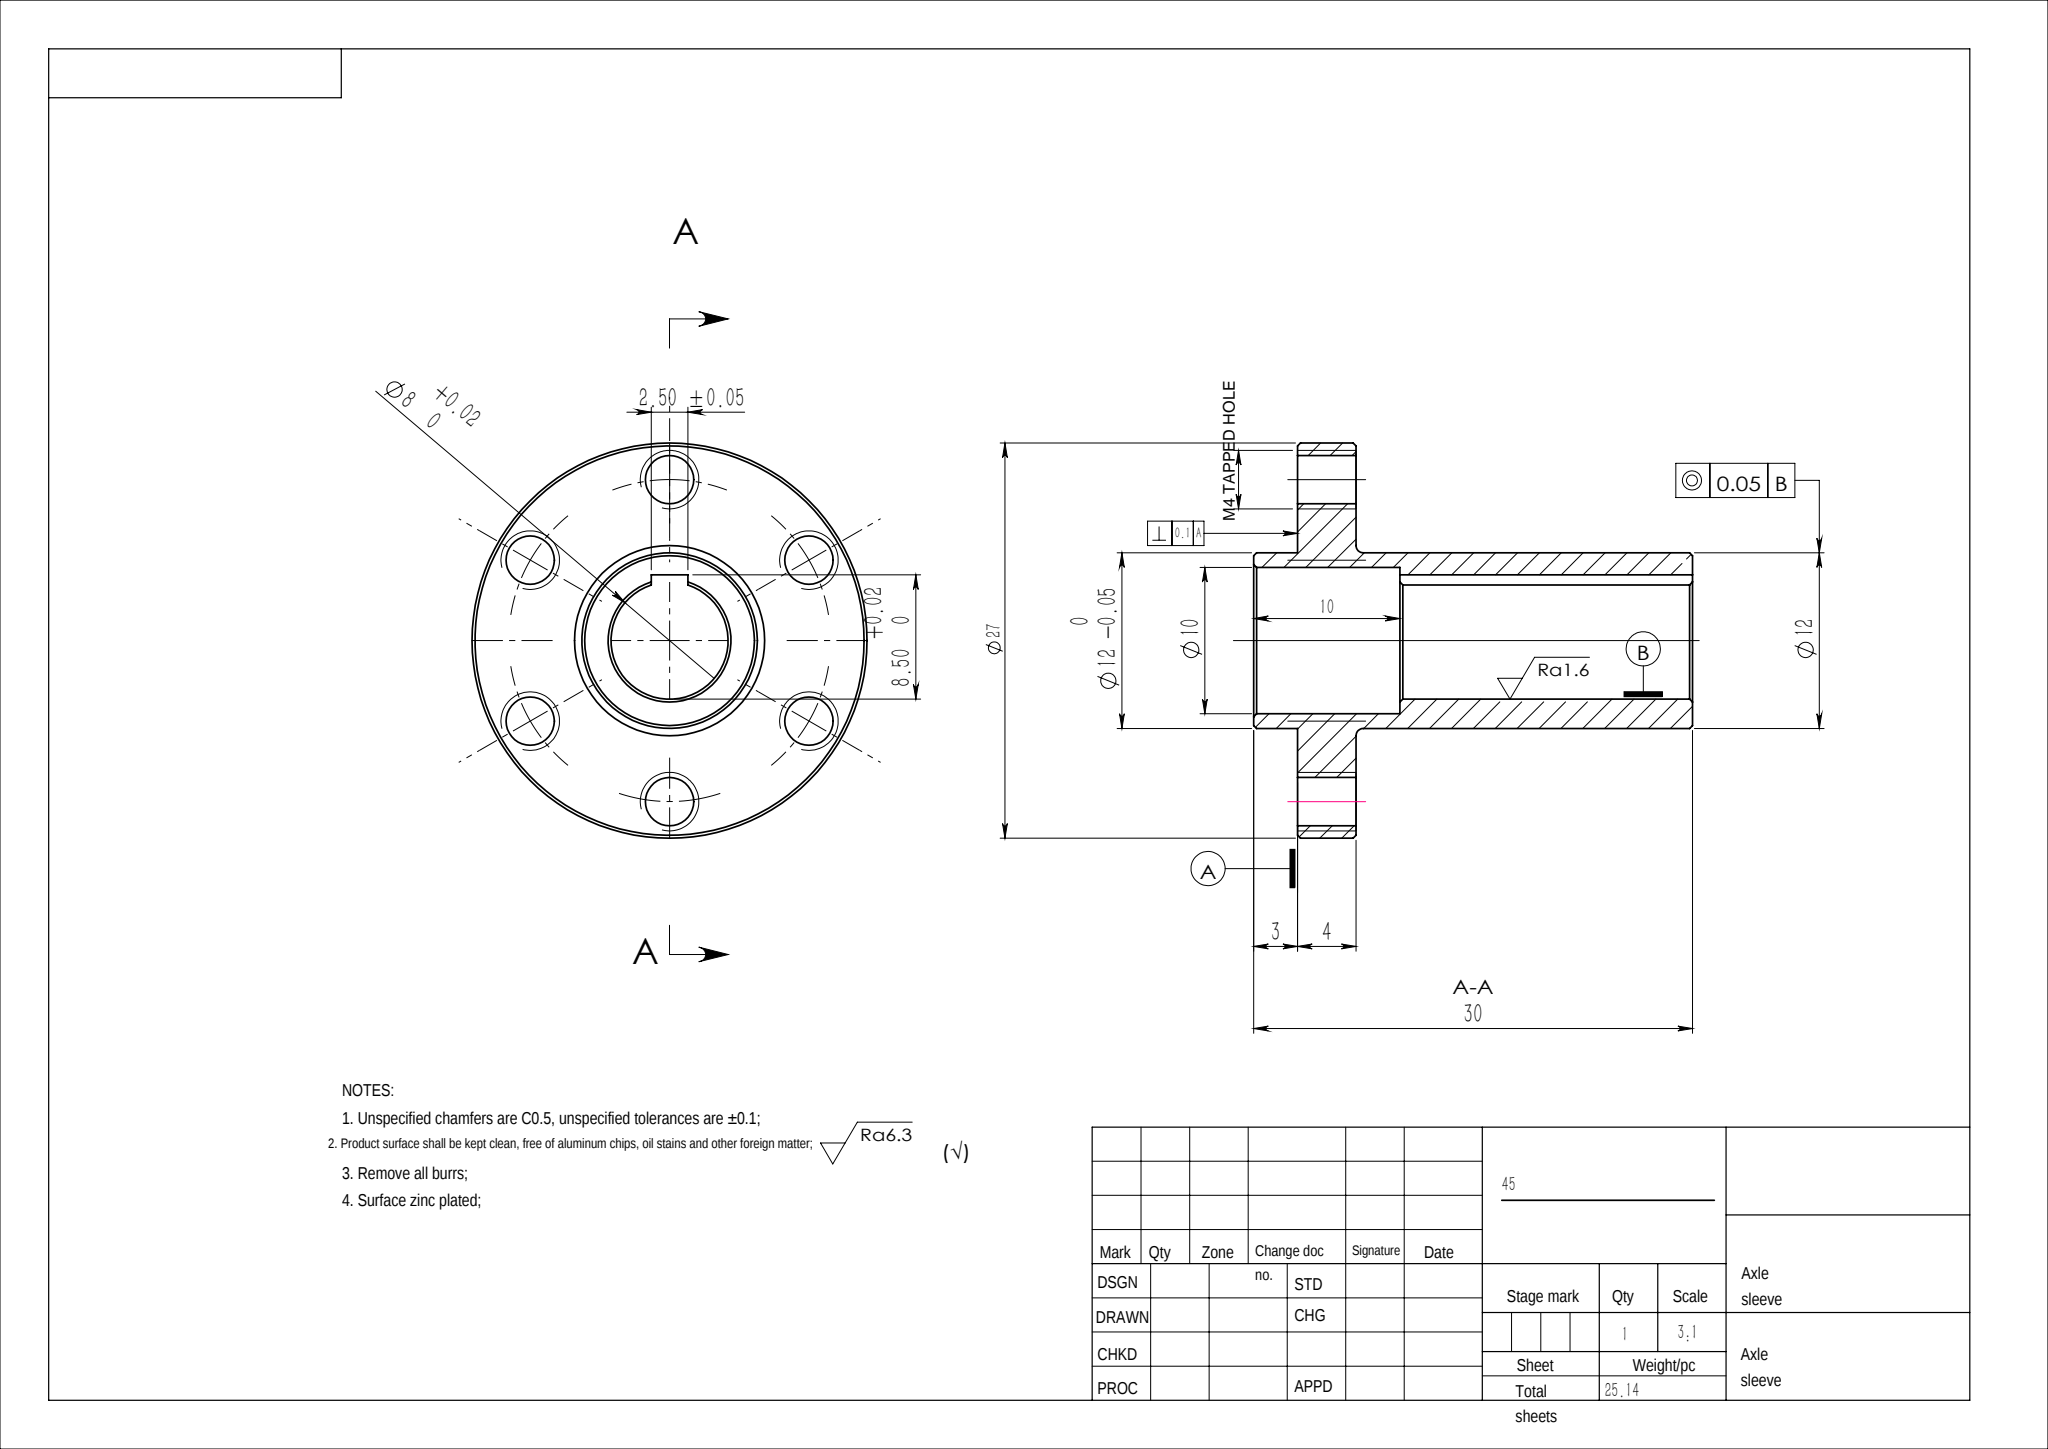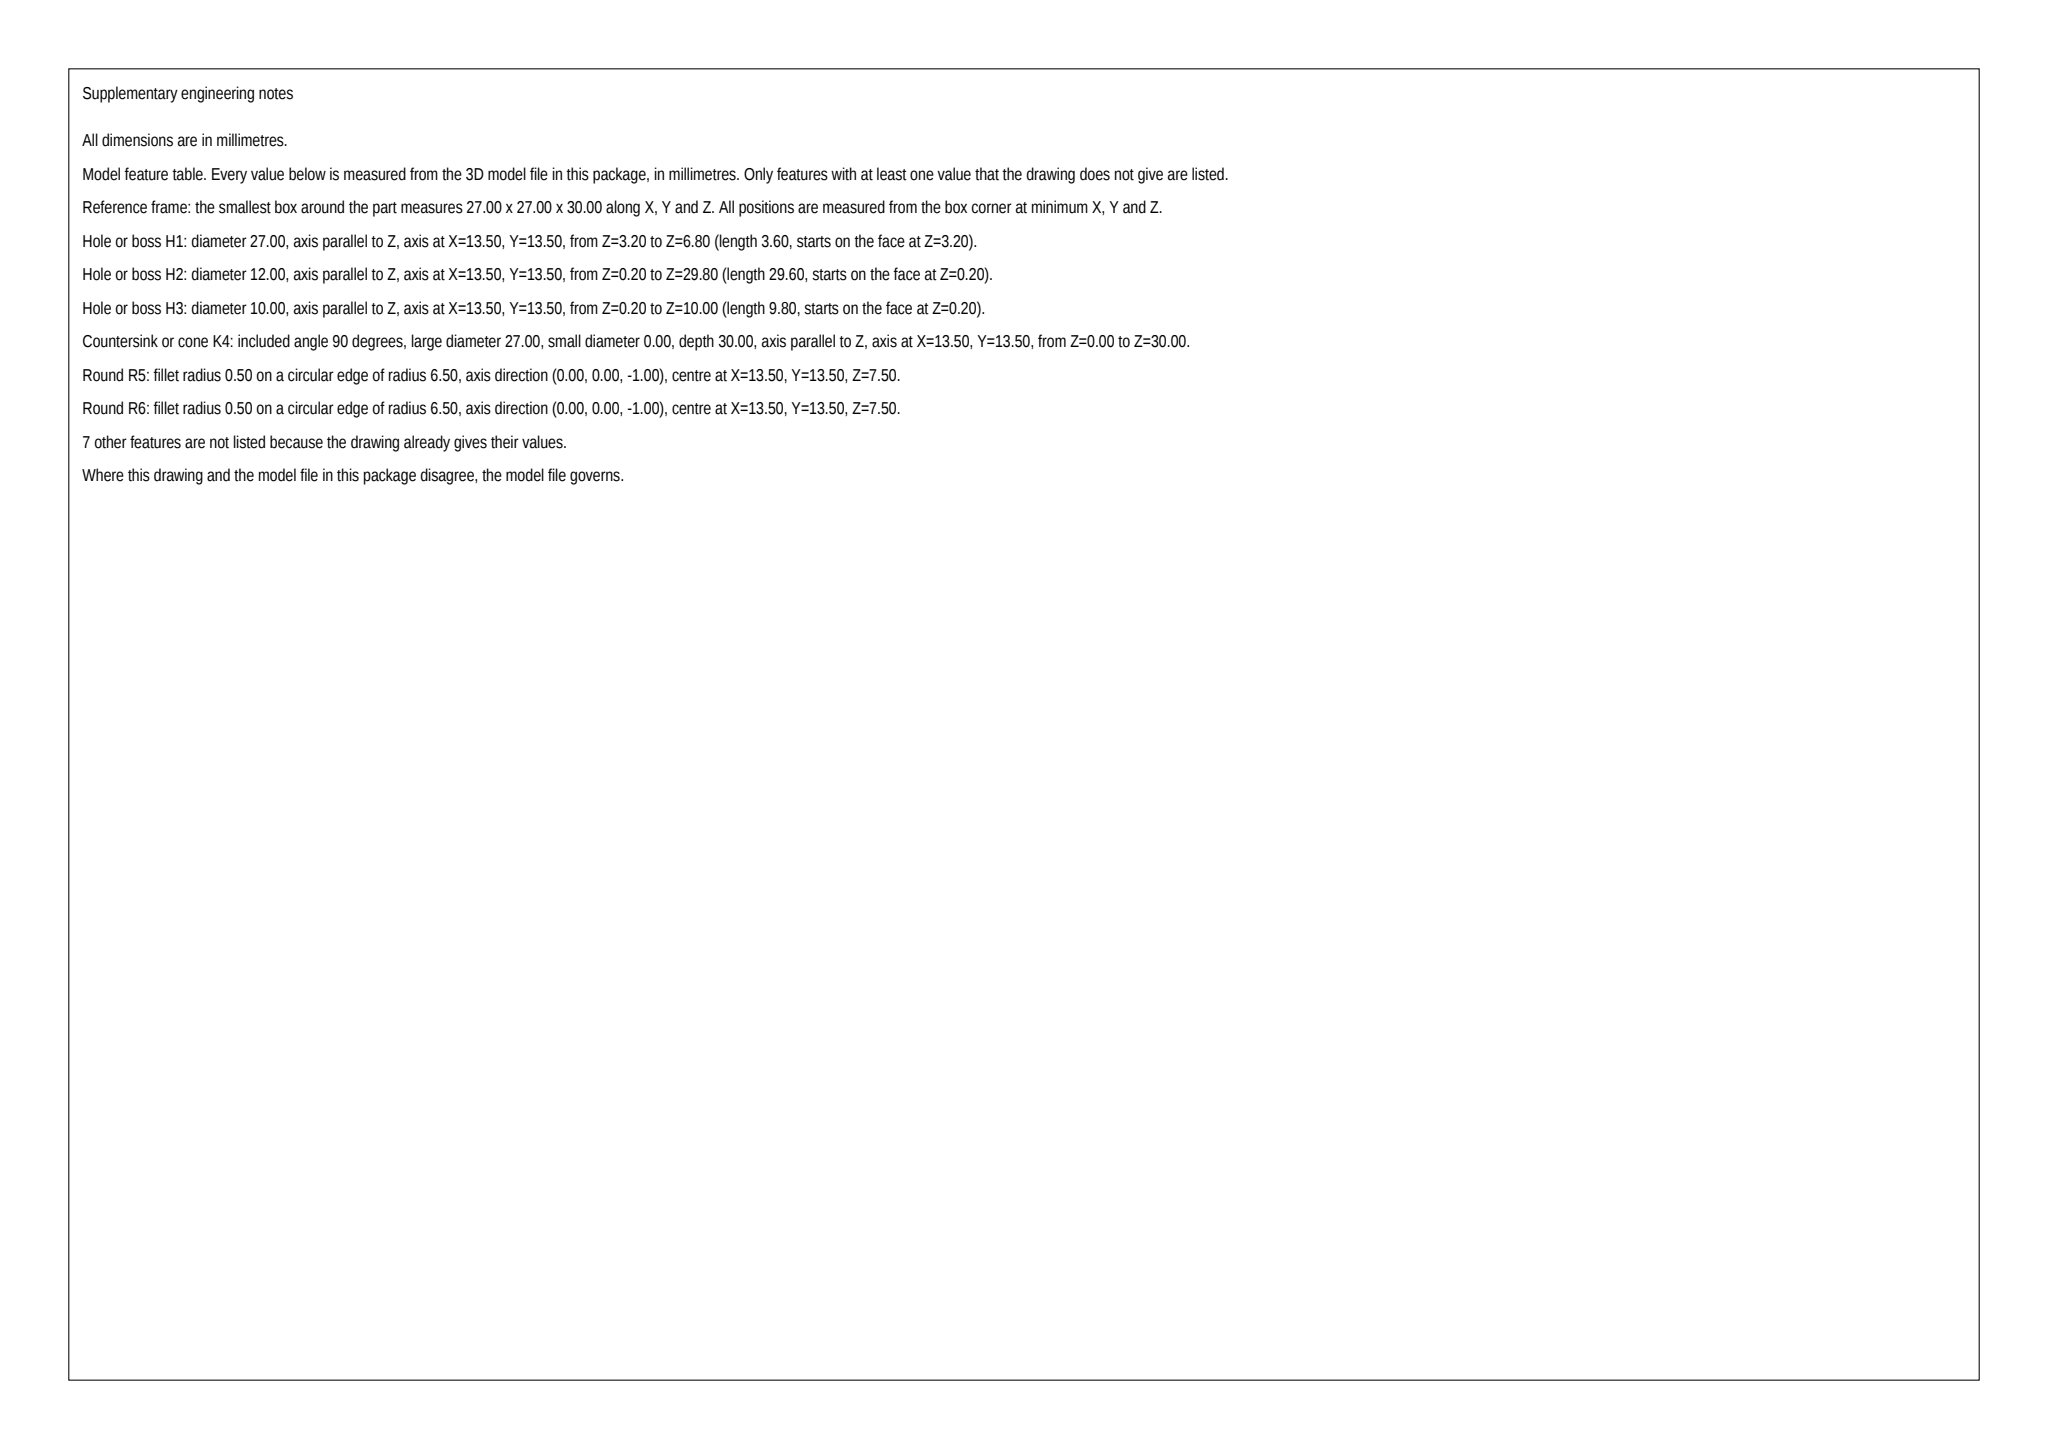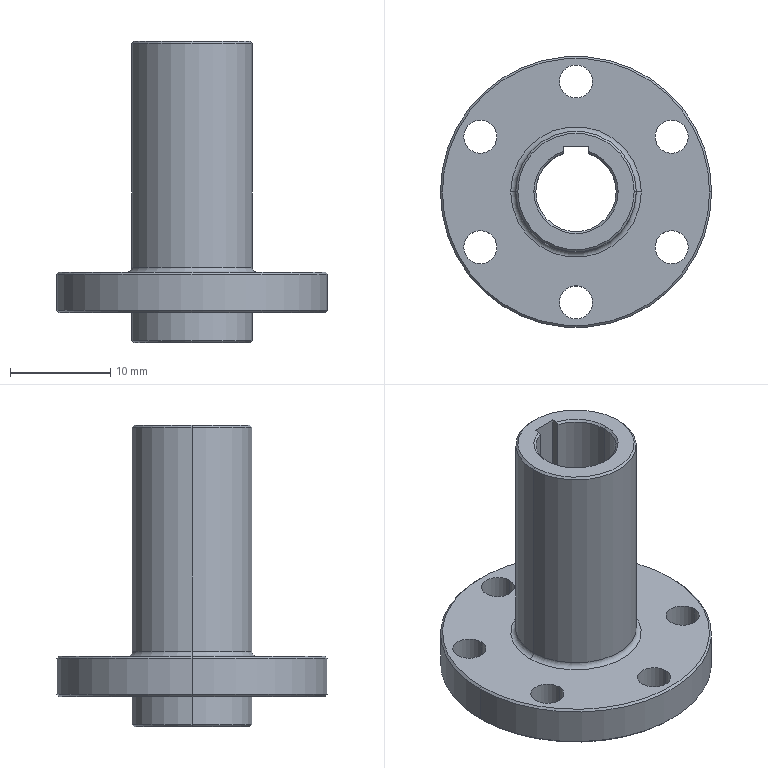Part | SolidWorks | mm | 1 solid | 49 faces | box 27 x 27 x 30 mm | volume 3202 mm3 | cylinder 23 | cone 16 | plane 8 | torus 2 | commonest cylinder face diameters 3.3 x12 12 x4 8 x3 10 x2 27 x2
build123d program:
from build123d import *

# Parameters (mm, degrees)
SKETCH4_W             = 21.152
SKETCH4_H             = 2.5
EXTRUDE3_DEPTH        = 1.25
SKETCH3_R             = 1.6
CUT_EXTRUDE1_DEPTH    = 30
CIRPATTERN1_COUNT     = 6
CHAMFER1_SIZE         = 0.2
M4_TAPPED_HOLE1_D     = 3.3
M4_TAPPED_HOLE1_DEPTH = 10.1
M4_TAPPED_HOLE1_TIP   = 0.9914


with BuildPart() as part:
    # Sketch1 → Revolve1 (revolve)
    with BuildSketch(Plane(origin=(0, 0, 0), x_dir=(1, 0, 0), z_dir=(0, 1, 0))):
        with BuildLine():
            Line((-6, 0), (-4, 0))
            Line((-4, 0), (-4, 20))
            Line((-4, 20), (-5, 20))
            Line((-5, 20), (-5, 30))
            Line((-5, 30), (-6, 30))
            Line((-6, 30), (-6, 27))
            Line((-6, 27), (-13.5, 27))
            Line((-13.5, 27), (-13.5, 23))
            Line((-13.5, 23), (-6.5, 23))
            ThreePointArc((-6.5, 23), (-6.146, 22.854), (-6, 22.5))
            Line((-6, 22.5), (-6, 0))
        make_face()
    revolve(axis=Axis((0, 0, -185.898), (0, 0, 1)))

    # Sketch4 → Extrude3 (cut, symmetric)
    with BuildSketch(Plane(origin=(0, 0, 0), x_dir=(0, 0, -1), z_dir=(1, 0, 0))):
        with Locations((10.576, 3.25)):
            Rectangle(SKETCH4_W, SKETCH4_H)
    extrude(amount=EXTRUDE3_DEPTH, both=True, mode=Mode.SUBTRACT)

    # Sketch3 → Cut-Extrude1 (cut)
    with BuildSketch(Plane(origin=(0, 0, -27), x_dir=(-1, 0, 0), z_dir=(0, 0, -1))):
        with Locations((0, 11)):
            Circle(SKETCH3_R)
    cut_extrude1 = extrude(amount=-CUT_EXTRUDE1_DEPTH, mode=Mode.SUBTRACT)

    # CirPattern1: Cut-Extrude1 ×6 about axis
    cirpattern1_axis = Axis((0, 0, 0), (0, 0, 1))
    for i in range(1, CIRPATTERN1_COUNT):
        add(cut_extrude1.rotate(cirpattern1_axis, i * 360 / CIRPATTERN1_COUNT), mode=Mode.SUBTRACT)

    # Chamfer1
    chamfer1_edges = [part.edges().sort_by_distance(p)[0] for p in [
        (6, 0, -30),
        (13.5, 0, -27),
        (13.5, 0, -23),
        (0, -4, 0),
        (0, -4, -20),
        (6, 0, 0),
        (5, 0, -30),
    ]]
    chamfer(chamfer1_edges, length=CHAMFER1_SIZE)

    # M4 Tapped Hole1
    with Locations(Plane(origin=(0, 0, -27), x_dir=(-1, 0, 0), z_dir=(0, 0, -1))):
        with Locations((0, 11), (-9.526, 5.5), (-9.526, -5.5), (0, -11), (9.526, -5.5), (9.526, 5.5)):
            Hole(M4_TAPPED_HOLE1_D / 2, depth=M4_TAPPED_HOLE1_DEPTH)
            with Locations((0, 0, -(M4_TAPPED_HOLE1_DEPTH + M4_TAPPED_HOLE1_TIP / 2))):  # 118° drill point
                Cone(0, M4_TAPPED_HOLE1_D / 2, M4_TAPPED_HOLE1_TIP, mode=Mode.SUBTRACT)


solid = part.part